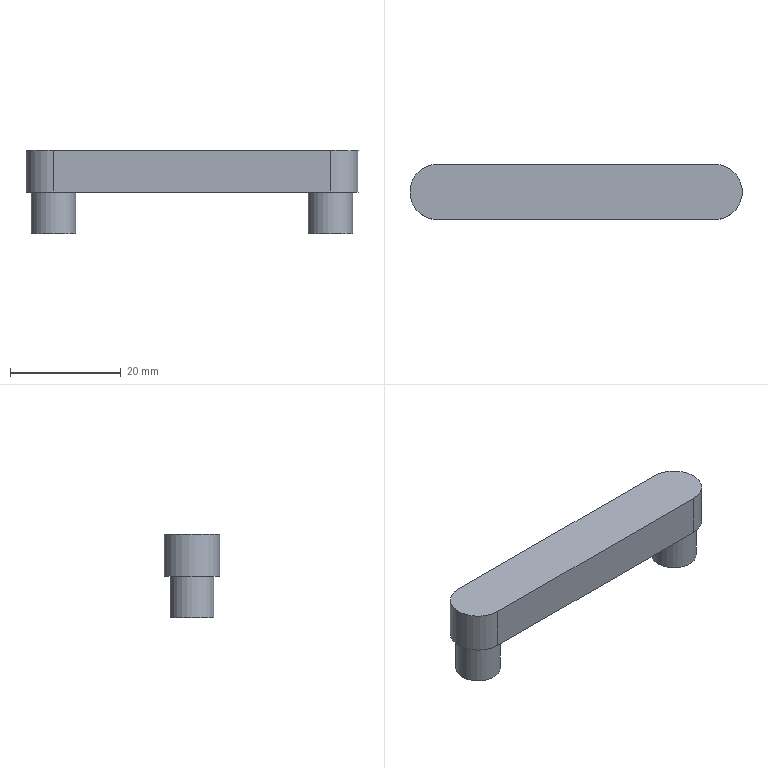Component | NX | STEERING_LINK | 1 solid | 10 faces | box 60 x 10 x 15 mm | volume 5093 mm3 | plane 6 | cylinder 4 | commonest cylinder face diameters 10 x2 8 x2
STEP:
#1=CARTESIAN_POINT('',(0.,0.,0.));
#2=DIRECTION('',(0.,0.,1.));
#3=DIRECTION('',(1.,0.,0.));
#4=AXIS2_PLACEMENT_3D('',#1,#2,#3);
#5=CARTESIAN_POINT('',(32.237,-74.16,30.));
#6=VERTEX_POINT('',#5);
#7=CARTESIAN_POINT('',(32.237,-64.16,30.));
#8=VERTEX_POINT('',#7);
#9=CARTESIAN_POINT('',(32.237,-69.16,30.));
#10=DIRECTION('',(0.,0.,-1.));
#11=DIRECTION('',(1.,0.,0.));
#12=AXIS2_PLACEMENT_3D('',#9,#10,#11);
#13=CIRCLE('',#12,5.);
#14=CARTESIAN_POINT('',(32.237,-69.16,22.5));
#15=DIRECTION('',(0.,0.,1.));
#16=DIRECTION('',(-1.,0.,0.));
#17=AXIS2_PLACEMENT_3D('',#14,#15,#16);
#18=CYLINDRICAL_SURFACE('',#17,5.);
#19=CARTESIAN_POINT('',(3.142,7.5));
#20=DIRECTION('',(-1.,0.));
#21=VECTOR('',#20,1.);
#22=LINE('',#19,#21);
#23=(GEOMETRIC_REPRESENTATION_CONTEXT(2)PARAMETRIC_REPRESENTATION_CONTEXT()REPRESENTATION_CONTEXT('',''));
#24=DEFINITIONAL_REPRESENTATION('',(#22),#23);
#25=PCURVE('',#18,#24);
#26=CARTESIAN_POINT('',(32.237,-69.16,30.));
#27=DIRECTION('',(0.,0.,-1.));
#28=DIRECTION('',(1.,0.,0.));
#29=AXIS2_PLACEMENT_3D('',#26,#27,#28);
#30=PLANE('',#29);
#31=CARTESIAN_POINT('',(0.,0.));
#32=DIRECTION('',(1.,0.));
#33=AXIS2_PLACEMENT_2D('',#31,#32);
#34=CIRCLE('',#33,5.);
#35=(GEOMETRIC_REPRESENTATION_CONTEXT(2)PARAMETRIC_REPRESENTATION_CONTEXT()REPRESENTATION_CONTEXT('',''));
#36=DEFINITIONAL_REPRESENTATION('',(#34),#35);
#37=PCURVE('',#30,#36);
#38=SURFACE_CURVE('',#13,(#25,#37),.PCURVE_S1.);
#39=EDGE_CURVE('',#6,#8,#38,.T.);
#40=ORIENTED_EDGE('',*,*,#39,.T.);
#41=CARTESIAN_POINT('',(32.237,-64.16,22.5));
#42=VERTEX_POINT('',#41);
#43=CARTESIAN_POINT('',(32.237,-64.16,22.5));
#44=DIRECTION('',(0.,0.,1.));
#45=VECTOR('',#44,1.);
#46=LINE('',#43,#45);
#47=CARTESIAN_POINT('',(-1.571,0.));
#48=DIRECTION('',(0.,1.));
#49=VECTOR('',#48,1.);
#50=LINE('',#47,#49);
#51=(GEOMETRIC_REPRESENTATION_CONTEXT(2)PARAMETRIC_REPRESENTATION_CONTEXT()REPRESENTATION_CONTEXT('',''));
#52=DEFINITIONAL_REPRESENTATION('',(#50),#51);
#53=PCURVE('',#18,#52);
#54=CARTESIAN_POINT('',(32.237,-64.16,22.5));
#55=DIRECTION('',(0.,-1.,0.));
#56=DIRECTION('',(0.,0.,-1.));
#57=AXIS2_PLACEMENT_3D('',#54,#55,#56);
#58=PLANE('',#57);
#59=CARTESIAN_POINT('',(0.,0.));
#60=DIRECTION('',(-1.,0.));
#61=VECTOR('',#60,1.);
#62=LINE('',#59,#61);
#63=(GEOMETRIC_REPRESENTATION_CONTEXT(2)PARAMETRIC_REPRESENTATION_CONTEXT()REPRESENTATION_CONTEXT('',''));
#64=DEFINITIONAL_REPRESENTATION('',(#62),#63);
#65=PCURVE('',#58,#64);
#66=SURFACE_CURVE('',#46,(#53,#65),.PCURVE_S1.);
#67=EDGE_CURVE('',#42,#8,#66,.T.);
#68=ORIENTED_EDGE('',*,*,#67,.F.);
#69=CARTESIAN_POINT('',(32.237,-74.16,22.5));
#70=VERTEX_POINT('',#69);
#71=CARTESIAN_POINT('',(32.237,-69.16,22.5));
#72=DIRECTION('',(0.,0.,-1.));
#73=DIRECTION('',(1.,0.,0.));
#74=AXIS2_PLACEMENT_3D('',#71,#72,#73);
#75=CIRCLE('',#74,5.);
#76=CARTESIAN_POINT('',(3.142,0.));
#77=DIRECTION('',(-1.,0.));
#78=VECTOR('',#77,1.);
#79=LINE('',#76,#78);
#80=(GEOMETRIC_REPRESENTATION_CONTEXT(2)PARAMETRIC_REPRESENTATION_CONTEXT()REPRESENTATION_CONTEXT('',''));
#81=DEFINITIONAL_REPRESENTATION('',(#79),#80);
#82=PCURVE('',#18,#81);
#83=CARTESIAN_POINT('',(32.237,-69.16,22.5));
#84=DIRECTION('',(0.,0.,-1.));
#85=DIRECTION('',(1.,0.,0.));
#86=AXIS2_PLACEMENT_3D('',#83,#84,#85);
#87=PLANE('',#86);
#88=CARTESIAN_POINT('',(0.,0.));
#89=DIRECTION('',(1.,0.));
#90=AXIS2_PLACEMENT_2D('',#88,#89);
#91=CIRCLE('',#90,5.);
#92=(GEOMETRIC_REPRESENTATION_CONTEXT(2)PARAMETRIC_REPRESENTATION_CONTEXT()REPRESENTATION_CONTEXT('',''));
#93=DEFINITIONAL_REPRESENTATION('',(#91),#92);
#94=PCURVE('',#87,#93);
#95=SURFACE_CURVE('',#75,(#82,#94),.PCURVE_S1.);
#96=EDGE_CURVE('',#70,#42,#95,.T.);
#97=ORIENTED_EDGE('',*,*,#96,.F.);
#98=CARTESIAN_POINT('',(32.237,-74.16,22.5));
#99=DIRECTION('',(0.,0.,1.));
#100=VECTOR('',#99,1.);
#101=LINE('',#98,#100);
#102=CARTESIAN_POINT('',(1.571,0.));
#103=DIRECTION('',(0.,1.));
#104=VECTOR('',#103,1.);
#105=LINE('',#102,#104);
#106=(GEOMETRIC_REPRESENTATION_CONTEXT(2)PARAMETRIC_REPRESENTATION_CONTEXT()REPRESENTATION_CONTEXT('',''));
#107=DEFINITIONAL_REPRESENTATION('',(#105),#106);
#108=PCURVE('',#18,#107);
#109=CARTESIAN_POINT('',(82.237,-74.16,22.5));
#110=DIRECTION('',(0.,1.,0.));
#111=DIRECTION('',(0.,0.,1.));
#112=AXIS2_PLACEMENT_3D('',#109,#110,#111);
#113=PLANE('',#112);
#114=CARTESIAN_POINT('',(0.,-50.));
#115=DIRECTION('',(1.,0.));
#116=VECTOR('',#115,1.);
#117=LINE('',#114,#116);
#118=(GEOMETRIC_REPRESENTATION_CONTEXT(2)PARAMETRIC_REPRESENTATION_CONTEXT()REPRESENTATION_CONTEXT('',''));
#119=DEFINITIONAL_REPRESENTATION('',(#117),#118);
#120=PCURVE('',#113,#119);
#121=SURFACE_CURVE('',#101,(#108,#120),.PCURVE_S1.);
#122=EDGE_CURVE('',#70,#6,#121,.T.);
#123=ORIENTED_EDGE('',*,*,#122,.T.);
#124=EDGE_LOOP('',(#40,#68,#97,#123));
#125=FACE_BOUND('',#124,.T.);
#126=ADVANCED_FACE('',(#125),#18,.T.);
#127=CARTESIAN_POINT('',(82.237,-64.16,30.));
#128=VERTEX_POINT('',#127);
#129=CARTESIAN_POINT('',(32.237,-64.16,30.));
#130=DIRECTION('',(1.,0.,0.));
#131=VECTOR('',#130,1.);
#132=LINE('',#129,#131);
#133=CARTESIAN_POINT('',(-7.5,0.));
#134=DIRECTION('',(0.,1.));
#135=VECTOR('',#134,1.);
#136=LINE('',#133,#135);
#137=(GEOMETRIC_REPRESENTATION_CONTEXT(2)PARAMETRIC_REPRESENTATION_CONTEXT()REPRESENTATION_CONTEXT('',''));
#138=DEFINITIONAL_REPRESENTATION('',(#136),#137);
#139=PCURVE('',#58,#138);
#140=CARTESIAN_POINT('',(0.,-5.));
#141=DIRECTION('',(1.,0.));
#142=VECTOR('',#141,1.);
#143=LINE('',#140,#142);
#144=(GEOMETRIC_REPRESENTATION_CONTEXT(2)PARAMETRIC_REPRESENTATION_CONTEXT()REPRESENTATION_CONTEXT('',''));
#145=DEFINITIONAL_REPRESENTATION('',(#143),#144);
#146=PCURVE('',#30,#145);
#147=SURFACE_CURVE('',#132,(#139,#146),.PCURVE_S1.);
#148=EDGE_CURVE('',#8,#128,#147,.T.);
#149=ORIENTED_EDGE('',*,*,#148,.T.);
#150=CARTESIAN_POINT('',(82.237,-64.16,22.5));
#151=VERTEX_POINT('',#150);
#152=CARTESIAN_POINT('',(82.237,-64.16,22.5));
#153=DIRECTION('',(0.,0.,1.));
#154=VECTOR('',#153,1.);
#155=LINE('',#152,#154);
#156=CARTESIAN_POINT('',(0.,50.));
#157=DIRECTION('',(-1.,0.));
#158=VECTOR('',#157,1.);
#159=LINE('',#156,#158);
#160=(GEOMETRIC_REPRESENTATION_CONTEXT(2)PARAMETRIC_REPRESENTATION_CONTEXT()REPRESENTATION_CONTEXT('',''));
#161=DEFINITIONAL_REPRESENTATION('',(#159),#160);
#162=PCURVE('',#58,#161);
#163=CARTESIAN_POINT('',(82.237,-69.16,22.5));
#164=DIRECTION('',(0.,0.,1.));
#165=DIRECTION('',(-1.,0.,0.));
#166=AXIS2_PLACEMENT_3D('',#163,#164,#165);
#167=CYLINDRICAL_SURFACE('',#166,5.);
#168=CARTESIAN_POINT('',(4.712,0.));
#169=DIRECTION('',(0.,1.));
#170=VECTOR('',#169,1.);
#171=LINE('',#168,#170);
#172=(GEOMETRIC_REPRESENTATION_CONTEXT(2)PARAMETRIC_REPRESENTATION_CONTEXT()REPRESENTATION_CONTEXT('',''));
#173=DEFINITIONAL_REPRESENTATION('',(#171),#172);
#174=PCURVE('',#167,#173);
#175=SURFACE_CURVE('',#155,(#162,#174),.PCURVE_S1.);
#176=EDGE_CURVE('',#151,#128,#175,.T.);
#177=ORIENTED_EDGE('',*,*,#176,.F.);
#178=CARTESIAN_POINT('',(32.237,-64.16,22.5));
#179=DIRECTION('',(1.,0.,0.));
#180=VECTOR('',#179,1.);
#181=LINE('',#178,#180);
#182=CARTESIAN_POINT('',(0.,0.));
#183=DIRECTION('',(0.,1.));
#184=VECTOR('',#183,1.);
#185=LINE('',#182,#184);
#186=(GEOMETRIC_REPRESENTATION_CONTEXT(2)PARAMETRIC_REPRESENTATION_CONTEXT()REPRESENTATION_CONTEXT('',''));
#187=DEFINITIONAL_REPRESENTATION('',(#185),#186);
#188=PCURVE('',#58,#187);
#189=CARTESIAN_POINT('',(0.,-5.));
#190=DIRECTION('',(1.,0.));
#191=VECTOR('',#190,1.);
#192=LINE('',#189,#191);
#193=(GEOMETRIC_REPRESENTATION_CONTEXT(2)PARAMETRIC_REPRESENTATION_CONTEXT()REPRESENTATION_CONTEXT('',''));
#194=DEFINITIONAL_REPRESENTATION('',(#192),#193);
#195=PCURVE('',#87,#194);
#196=SURFACE_CURVE('',#181,(#188,#195),.PCURVE_S1.);
#197=EDGE_CURVE('',#42,#151,#196,.T.);
#198=ORIENTED_EDGE('',*,*,#197,.F.);
#199=ORIENTED_EDGE('',*,*,#67,.T.);
#200=EDGE_LOOP('',(#149,#177,#198,#199));
#201=FACE_BOUND('',#200,.T.);
#202=ADVANCED_FACE('',(#201),#58,.F.);
#203=CARTESIAN_POINT('',(82.237,-74.16,30.));
#204=VERTEX_POINT('',#203);
#205=CARTESIAN_POINT('',(82.237,-69.16,30.));
#206=DIRECTION('',(0.,0.,-1.));
#207=DIRECTION('',(1.,0.,0.));
#208=AXIS2_PLACEMENT_3D('',#205,#206,#207);
#209=CIRCLE('',#208,5.);
#210=CARTESIAN_POINT('',(9.425,7.5));
#211=DIRECTION('',(-1.,0.));
#212=VECTOR('',#211,1.);
#213=LINE('',#210,#212);
#214=(GEOMETRIC_REPRESENTATION_CONTEXT(2)PARAMETRIC_REPRESENTATION_CONTEXT()REPRESENTATION_CONTEXT('',''));
#215=DEFINITIONAL_REPRESENTATION('',(#213),#214);
#216=PCURVE('',#167,#215);
#217=CARTESIAN_POINT('',(50.,0.));
#218=DIRECTION('',(1.,0.));
#219=AXIS2_PLACEMENT_2D('',#217,#218);
#220=CIRCLE('',#219,5.);
#221=(GEOMETRIC_REPRESENTATION_CONTEXT(2)PARAMETRIC_REPRESENTATION_CONTEXT()REPRESENTATION_CONTEXT('',''));
#222=DEFINITIONAL_REPRESENTATION('',(#220),#221);
#223=PCURVE('',#30,#222);
#224=SURFACE_CURVE('',#209,(#216,#223),.PCURVE_S1.);
#225=EDGE_CURVE('',#128,#204,#224,.T.);
#226=ORIENTED_EDGE('',*,*,#225,.T.);
#227=CARTESIAN_POINT('',(82.237,-74.16,22.5));
#228=VERTEX_POINT('',#227);
#229=CARTESIAN_POINT('',(82.237,-74.16,22.5));
#230=DIRECTION('',(0.,0.,1.));
#231=VECTOR('',#230,1.);
#232=LINE('',#229,#231);
#233=CARTESIAN_POINT('',(1.571,0.));
#234=DIRECTION('',(0.,1.));
#235=VECTOR('',#234,1.);
#236=LINE('',#233,#235);
#237=(GEOMETRIC_REPRESENTATION_CONTEXT(2)PARAMETRIC_REPRESENTATION_CONTEXT()REPRESENTATION_CONTEXT('',''));
#238=DEFINITIONAL_REPRESENTATION('',(#236),#237);
#239=PCURVE('',#167,#238);
#240=CARTESIAN_POINT('',(0.,0.));
#241=DIRECTION('',(1.,0.));
#242=VECTOR('',#241,1.);
#243=LINE('',#240,#242);
#244=(GEOMETRIC_REPRESENTATION_CONTEXT(2)PARAMETRIC_REPRESENTATION_CONTEXT()REPRESENTATION_CONTEXT('',''));
#245=DEFINITIONAL_REPRESENTATION('',(#243),#244);
#246=PCURVE('',#113,#245);
#247=SURFACE_CURVE('',#232,(#239,#246),.PCURVE_S1.);
#248=EDGE_CURVE('',#228,#204,#247,.T.);
#249=ORIENTED_EDGE('',*,*,#248,.F.);
#250=CARTESIAN_POINT('',(82.237,-69.16,22.5));
#251=DIRECTION('',(0.,0.,-1.));
#252=DIRECTION('',(1.,0.,0.));
#253=AXIS2_PLACEMENT_3D('',#250,#251,#252);
#254=CIRCLE('',#253,5.);
#255=CARTESIAN_POINT('',(9.425,0.));
#256=DIRECTION('',(-1.,0.));
#257=VECTOR('',#256,1.);
#258=LINE('',#255,#257);
#259=(GEOMETRIC_REPRESENTATION_CONTEXT(2)PARAMETRIC_REPRESENTATION_CONTEXT()REPRESENTATION_CONTEXT('',''));
#260=DEFINITIONAL_REPRESENTATION('',(#258),#259);
#261=PCURVE('',#167,#260);
#262=CARTESIAN_POINT('',(50.,0.));
#263=DIRECTION('',(1.,0.));
#264=AXIS2_PLACEMENT_2D('',#262,#263);
#265=CIRCLE('',#264,5.);
#266=(GEOMETRIC_REPRESENTATION_CONTEXT(2)PARAMETRIC_REPRESENTATION_CONTEXT()REPRESENTATION_CONTEXT('',''));
#267=DEFINITIONAL_REPRESENTATION('',(#265),#266);
#268=PCURVE('',#87,#267);
#269=SURFACE_CURVE('',#254,(#261,#268),.PCURVE_S1.);
#270=EDGE_CURVE('',#151,#228,#269,.T.);
#271=ORIENTED_EDGE('',*,*,#270,.F.);
#272=ORIENTED_EDGE('',*,*,#176,.T.);
#273=EDGE_LOOP('',(#226,#249,#271,#272));
#274=FACE_BOUND('',#273,.T.);
#275=ADVANCED_FACE('',(#274),#167,.T.);
#276=CARTESIAN_POINT('',(82.237,-74.16,30.));
#277=DIRECTION('',(-1.,0.,0.));
#278=VECTOR('',#277,1.);
#279=LINE('',#276,#278);
#280=CARTESIAN_POINT('',(7.5,0.));
#281=DIRECTION('',(0.,-1.));
#282=VECTOR('',#281,1.);
#283=LINE('',#280,#282);
#284=(GEOMETRIC_REPRESENTATION_CONTEXT(2)PARAMETRIC_REPRESENTATION_CONTEXT()REPRESENTATION_CONTEXT('',''));
#285=DEFINITIONAL_REPRESENTATION('',(#283),#284);
#286=PCURVE('',#113,#285);
#287=CARTESIAN_POINT('',(50.,5.));
#288=DIRECTION('',(-1.,0.));
#289=VECTOR('',#288,1.);
#290=LINE('',#287,#289);
#291=(GEOMETRIC_REPRESENTATION_CONTEXT(2)PARAMETRIC_REPRESENTATION_CONTEXT()REPRESENTATION_CONTEXT('',''));
#292=DEFINITIONAL_REPRESENTATION('',(#290),#291);
#293=PCURVE('',#30,#292);
#294=SURFACE_CURVE('',#279,(#286,#293),.PCURVE_S1.);
#295=EDGE_CURVE('',#204,#6,#294,.T.);
#296=ORIENTED_EDGE('',*,*,#295,.T.);
#297=ORIENTED_EDGE('',*,*,#122,.F.);
#298=CARTESIAN_POINT('',(82.237,-74.16,22.5));
#299=DIRECTION('',(-1.,0.,0.));
#300=VECTOR('',#299,1.);
#301=LINE('',#298,#300);
#302=CARTESIAN_POINT('',(0.,0.));
#303=DIRECTION('',(0.,-1.));
#304=VECTOR('',#303,1.);
#305=LINE('',#302,#304);
#306=(GEOMETRIC_REPRESENTATION_CONTEXT(2)PARAMETRIC_REPRESENTATION_CONTEXT()REPRESENTATION_CONTEXT('',''));
#307=DEFINITIONAL_REPRESENTATION('',(#305),#306);
#308=PCURVE('',#113,#307);
#309=CARTESIAN_POINT('',(50.,5.));
#310=DIRECTION('',(-1.,0.));
#311=VECTOR('',#310,1.);
#312=LINE('',#309,#311);
#313=(GEOMETRIC_REPRESENTATION_CONTEXT(2)PARAMETRIC_REPRESENTATION_CONTEXT()REPRESENTATION_CONTEXT('',''));
#314=DEFINITIONAL_REPRESENTATION('',(#312),#313);
#315=PCURVE('',#87,#314);
#316=SURFACE_CURVE('',#301,(#308,#315),.PCURVE_S1.);
#317=EDGE_CURVE('',#228,#70,#316,.T.);
#318=ORIENTED_EDGE('',*,*,#317,.F.);
#319=ORIENTED_EDGE('',*,*,#248,.T.);
#320=EDGE_LOOP('',(#296,#297,#318,#319));
#321=FACE_BOUND('',#320,.T.);
#322=ADVANCED_FACE('',(#321),#113,.F.);
#323=CARTESIAN_POINT('',(36.237,-69.16,22.5));
#324=VERTEX_POINT('',#323);
#325=CARTESIAN_POINT('',(32.237,-69.16,22.5));
#326=DIRECTION('',(0.,0.,-1.));
#327=DIRECTION('',(1.,0.,0.));
#328=AXIS2_PLACEMENT_3D('',#325,#326,#327);
#329=CIRCLE('',#328,4.);
#330=CARTESIAN_POINT('',(0.,0.));
#331=DIRECTION('',(1.,0.));
#332=AXIS2_PLACEMENT_2D('',#330,#331);
#333=CIRCLE('',#332,4.);
#334=(GEOMETRIC_REPRESENTATION_CONTEXT(2)PARAMETRIC_REPRESENTATION_CONTEXT()REPRESENTATION_CONTEXT('',''));
#335=DEFINITIONAL_REPRESENTATION('',(#333),#334);
#336=PCURVE('',#87,#335);
#337=CARTESIAN_POINT('',(32.237,-69.16,15.));
#338=DIRECTION('',(0.,0.,1.));
#339=DIRECTION('',(-1.,0.,0.));
#340=AXIS2_PLACEMENT_3D('',#337,#338,#339);
#341=CYLINDRICAL_SURFACE('',#340,4.);
#342=CARTESIAN_POINT('',(9.425,7.5));
#343=DIRECTION('',(-1.,0.));
#344=VECTOR('',#343,1.);
#345=LINE('',#342,#344);
#346=(GEOMETRIC_REPRESENTATION_CONTEXT(2)PARAMETRIC_REPRESENTATION_CONTEXT()REPRESENTATION_CONTEXT('',''));
#347=DEFINITIONAL_REPRESENTATION('',(#345),#346);
#348=PCURVE('',#341,#347);
#349=SURFACE_CURVE('',#329,(#336,#348),.PCURVE_S1.);
#350=EDGE_CURVE('',#324,#324,#349,.T.);
#351=ORIENTED_EDGE('',*,*,#350,.F.);
#352=EDGE_LOOP('',(#351));
#353=FACE_BOUND('',#352,.T.);
#354=CARTESIAN_POINT('',(86.237,-69.16,22.5));
#355=VERTEX_POINT('',#354);
#356=CARTESIAN_POINT('',(82.237,-69.16,22.5));
#357=DIRECTION('',(0.,0.,-1.));
#358=DIRECTION('',(1.,0.,0.));
#359=AXIS2_PLACEMENT_3D('',#356,#357,#358);
#360=CIRCLE('',#359,4.);
#361=CARTESIAN_POINT('',(50.,0.));
#362=DIRECTION('',(1.,0.));
#363=AXIS2_PLACEMENT_2D('',#361,#362);
#364=CIRCLE('',#363,4.);
#365=(GEOMETRIC_REPRESENTATION_CONTEXT(2)PARAMETRIC_REPRESENTATION_CONTEXT()REPRESENTATION_CONTEXT('',''));
#366=DEFINITIONAL_REPRESENTATION('',(#364),#365);
#367=PCURVE('',#87,#366);
#368=CARTESIAN_POINT('',(82.237,-69.16,15.));
#369=DIRECTION('',(0.,0.,1.));
#370=DIRECTION('',(-1.,0.,0.));
#371=AXIS2_PLACEMENT_3D('',#368,#369,#370);
#372=CYLINDRICAL_SURFACE('',#371,4.);
#373=CARTESIAN_POINT('',(9.425,7.5));
#374=DIRECTION('',(-1.,0.));
#375=VECTOR('',#374,1.);
#376=LINE('',#373,#375);
#377=(GEOMETRIC_REPRESENTATION_CONTEXT(2)PARAMETRIC_REPRESENTATION_CONTEXT()REPRESENTATION_CONTEXT('',''));
#378=DEFINITIONAL_REPRESENTATION('',(#376),#377);
#379=PCURVE('',#372,#378);
#380=SURFACE_CURVE('',#360,(#367,#379),.PCURVE_S1.);
#381=EDGE_CURVE('',#355,#355,#380,.T.);
#382=ORIENTED_EDGE('',*,*,#381,.F.);
#383=EDGE_LOOP('',(#382));
#384=FACE_BOUND('',#383,.T.);
#385=ORIENTED_EDGE('',*,*,#96,.T.);
#386=ORIENTED_EDGE('',*,*,#197,.T.);
#387=ORIENTED_EDGE('',*,*,#270,.T.);
#388=ORIENTED_EDGE('',*,*,#317,.T.);
#389=EDGE_LOOP('',(#385,#386,#387,#388));
#390=FACE_BOUND('',#389,.T.);
#391=ADVANCED_FACE('',(#353,#384,#390),#87,.T.);
#392=ORIENTED_EDGE('',*,*,#39,.F.);
#393=ORIENTED_EDGE('',*,*,#295,.F.);
#394=ORIENTED_EDGE('',*,*,#225,.F.);
#395=ORIENTED_EDGE('',*,*,#148,.F.);
#396=EDGE_LOOP('',(#392,#393,#394,#395));
#397=FACE_BOUND('',#396,.T.);
#398=ADVANCED_FACE('',(#397),#30,.F.);
#399=CARTESIAN_POINT('',(86.237,-69.16,15.));
#400=VERTEX_POINT('',#399);
#401=CARTESIAN_POINT('',(82.237,-69.16,15.));
#402=DIRECTION('',(0.,0.,-1.));
#403=DIRECTION('',(1.,0.,0.));
#404=AXIS2_PLACEMENT_3D('',#401,#402,#403);
#405=CIRCLE('',#404,4.);
#406=CARTESIAN_POINT('',(9.425,0.));
#407=DIRECTION('',(-1.,0.));
#408=VECTOR('',#407,1.);
#409=LINE('',#406,#408);
#410=(GEOMETRIC_REPRESENTATION_CONTEXT(2)PARAMETRIC_REPRESENTATION_CONTEXT()REPRESENTATION_CONTEXT('',''));
#411=DEFINITIONAL_REPRESENTATION('',(#409),#410);
#412=PCURVE('',#372,#411);
#413=CARTESIAN_POINT('',(82.237,-69.16,15.));
#414=DIRECTION('',(0.,0.,-1.));
#415=DIRECTION('',(1.,0.,0.));
#416=AXIS2_PLACEMENT_3D('',#413,#414,#415);
#417=PLANE('',#416);
#418=CARTESIAN_POINT('',(0.,0.));
#419=DIRECTION('',(1.,0.));
#420=AXIS2_PLACEMENT_2D('',#418,#419);
#421=CIRCLE('',#420,4.);
#422=(GEOMETRIC_REPRESENTATION_CONTEXT(2)PARAMETRIC_REPRESENTATION_CONTEXT()REPRESENTATION_CONTEXT('',''));
#423=DEFINITIONAL_REPRESENTATION('',(#421),#422);
#424=PCURVE('',#417,#423);
#425=SURFACE_CURVE('',#405,(#412,#424),.PCURVE_S1.);
#426=EDGE_CURVE('',#400,#400,#425,.T.);
#427=ORIENTED_EDGE('',*,*,#426,.F.);
#428=CARTESIAN_POINT('',(86.237,-69.16,15.));
#429=CARTESIAN_POINT('',(86.237,-69.16,22.5));
#430=B_SPLINE_CURVE_WITH_KNOTS('',1,(#428,#429),.UNSPECIFIED.,.F.,.F.,(2,2),(0.,7.5),.PIECEWISE_BEZIER_KNOTS.);
#431=CARTESIAN_POINT('',(9.425,0.));
#432=DIRECTION('',(0.,1.));
#433=VECTOR('',#432,1.);
#434=LINE('',#431,#433);
#435=(GEOMETRIC_REPRESENTATION_CONTEXT(2)PARAMETRIC_REPRESENTATION_CONTEXT()REPRESENTATION_CONTEXT('',''));
#436=DEFINITIONAL_REPRESENTATION('',(#434),#435);
#437=PCURVE('',#372,#436);
#438=CARTESIAN_POINT('',(3.142,0.));
#439=DIRECTION('',(0.,1.));
#440=VECTOR('',#439,1.);
#441=LINE('',#438,#440);
#442=(GEOMETRIC_REPRESENTATION_CONTEXT(2)PARAMETRIC_REPRESENTATION_CONTEXT()REPRESENTATION_CONTEXT('',''));
#443=DEFINITIONAL_REPRESENTATION('',(#441),#442);
#444=PCURVE('',#372,#443);
#445=SEAM_CURVE('',#430,(#437,#444),.PCURVE_S1.);
#446=EDGE_CURVE('',#400,#355,#445,.T.);
#447=ORIENTED_EDGE('',*,*,#446,.T.);
#448=ORIENTED_EDGE('',*,*,#381,.T.);
#449=ORIENTED_EDGE('',*,*,#446,.F.);
#450=EDGE_LOOP('',(#427,#447,#448,#449));
#451=FACE_BOUND('',#450,.T.);
#452=ADVANCED_FACE('',(#451),#372,.T.);
#453=ORIENTED_EDGE('',*,*,#426,.T.);
#454=EDGE_LOOP('',(#453));
#455=FACE_BOUND('',#454,.T.);
#456=ADVANCED_FACE('',(#455),#417,.T.);
#457=CARTESIAN_POINT('',(36.237,-69.16,15.));
#458=VERTEX_POINT('',#457);
#459=CARTESIAN_POINT('',(32.237,-69.16,15.));
#460=DIRECTION('',(0.,0.,-1.));
#461=DIRECTION('',(1.,0.,0.));
#462=AXIS2_PLACEMENT_3D('',#459,#460,#461);
#463=CIRCLE('',#462,4.);
#464=CARTESIAN_POINT('',(9.425,0.));
#465=DIRECTION('',(-1.,0.));
#466=VECTOR('',#465,1.);
#467=LINE('',#464,#466);
#468=(GEOMETRIC_REPRESENTATION_CONTEXT(2)PARAMETRIC_REPRESENTATION_CONTEXT()REPRESENTATION_CONTEXT('',''));
#469=DEFINITIONAL_REPRESENTATION('',(#467),#468);
#470=PCURVE('',#341,#469);
#471=CARTESIAN_POINT('',(32.237,-69.16,15.));
#472=DIRECTION('',(0.,0.,-1.));
#473=DIRECTION('',(1.,0.,0.));
#474=AXIS2_PLACEMENT_3D('',#471,#472,#473);
#475=PLANE('',#474);
#476=CARTESIAN_POINT('',(0.,0.));
#477=DIRECTION('',(1.,0.));
#478=AXIS2_PLACEMENT_2D('',#476,#477);
#479=CIRCLE('',#478,4.);
#480=(GEOMETRIC_REPRESENTATION_CONTEXT(2)PARAMETRIC_REPRESENTATION_CONTEXT()REPRESENTATION_CONTEXT('',''));
#481=DEFINITIONAL_REPRESENTATION('',(#479),#480);
#482=PCURVE('',#475,#481);
#483=SURFACE_CURVE('',#463,(#470,#482),.PCURVE_S1.);
#484=EDGE_CURVE('',#458,#458,#483,.T.);
#485=ORIENTED_EDGE('',*,*,#484,.F.);
#486=CARTESIAN_POINT('',(36.237,-69.16,15.));
#487=CARTESIAN_POINT('',(36.237,-69.16,22.5));
#488=B_SPLINE_CURVE_WITH_KNOTS('',1,(#486,#487),.UNSPECIFIED.,.F.,.F.,(2,2),(0.,7.5),.PIECEWISE_BEZIER_KNOTS.);
#489=CARTESIAN_POINT('',(9.425,0.));
#490=DIRECTION('',(0.,1.));
#491=VECTOR('',#490,1.);
#492=LINE('',#489,#491);
#493=(GEOMETRIC_REPRESENTATION_CONTEXT(2)PARAMETRIC_REPRESENTATION_CONTEXT()REPRESENTATION_CONTEXT('',''));
#494=DEFINITIONAL_REPRESENTATION('',(#492),#493);
#495=PCURVE('',#341,#494);
#496=CARTESIAN_POINT('',(3.142,0.));
#497=DIRECTION('',(0.,1.));
#498=VECTOR('',#497,1.);
#499=LINE('',#496,#498);
#500=(GEOMETRIC_REPRESENTATION_CONTEXT(2)PARAMETRIC_REPRESENTATION_CONTEXT()REPRESENTATION_CONTEXT('',''));
#501=DEFINITIONAL_REPRESENTATION('',(#499),#500);
#502=PCURVE('',#341,#501);
#503=SEAM_CURVE('',#488,(#495,#502),.PCURVE_S1.);
#504=EDGE_CURVE('',#458,#324,#503,.T.);
#505=ORIENTED_EDGE('',*,*,#504,.T.);
#506=ORIENTED_EDGE('',*,*,#350,.T.);
#507=ORIENTED_EDGE('',*,*,#504,.F.);
#508=EDGE_LOOP('',(#485,#505,#506,#507));
#509=FACE_BOUND('',#508,.T.);
#510=ADVANCED_FACE('',(#509),#341,.T.);
#511=ORIENTED_EDGE('',*,*,#484,.T.);
#512=EDGE_LOOP('',(#511));
#513=FACE_BOUND('',#512,.T.);
#514=ADVANCED_FACE('',(#513),#475,.T.);
#515=CLOSED_SHELL('',(#126,#202,#275,#322,#391,#398,#452,#456,#510,#514));
#516=MANIFOLD_SOLID_BREP('',#515);
#517=(LENGTH_UNIT()NAMED_UNIT(*)SI_UNIT(.MILLI.,.METRE.));
#518=UNCERTAINTY_MEASURE_WITH_UNIT(LENGTH_MEASURE(0.000002),#517,'','');
#519=(NAMED_UNIT(*)PLANE_ANGLE_UNIT()SI_UNIT($,.RADIAN.));
#520=(NAMED_UNIT(*)SI_UNIT($,.STERADIAN.)SOLID_ANGLE_UNIT());
#521=(GEOMETRIC_REPRESENTATION_CONTEXT(3)GLOBAL_UNCERTAINTY_ASSIGNED_CONTEXT((#518))GLOBAL_UNIT_ASSIGNED_CONTEXT((#517,#519,#520))REPRESENTATION_CONTEXT('',''));
#522=ADVANCED_BREP_SHAPE_REPRESENTATION('',(#4,#516),#521);